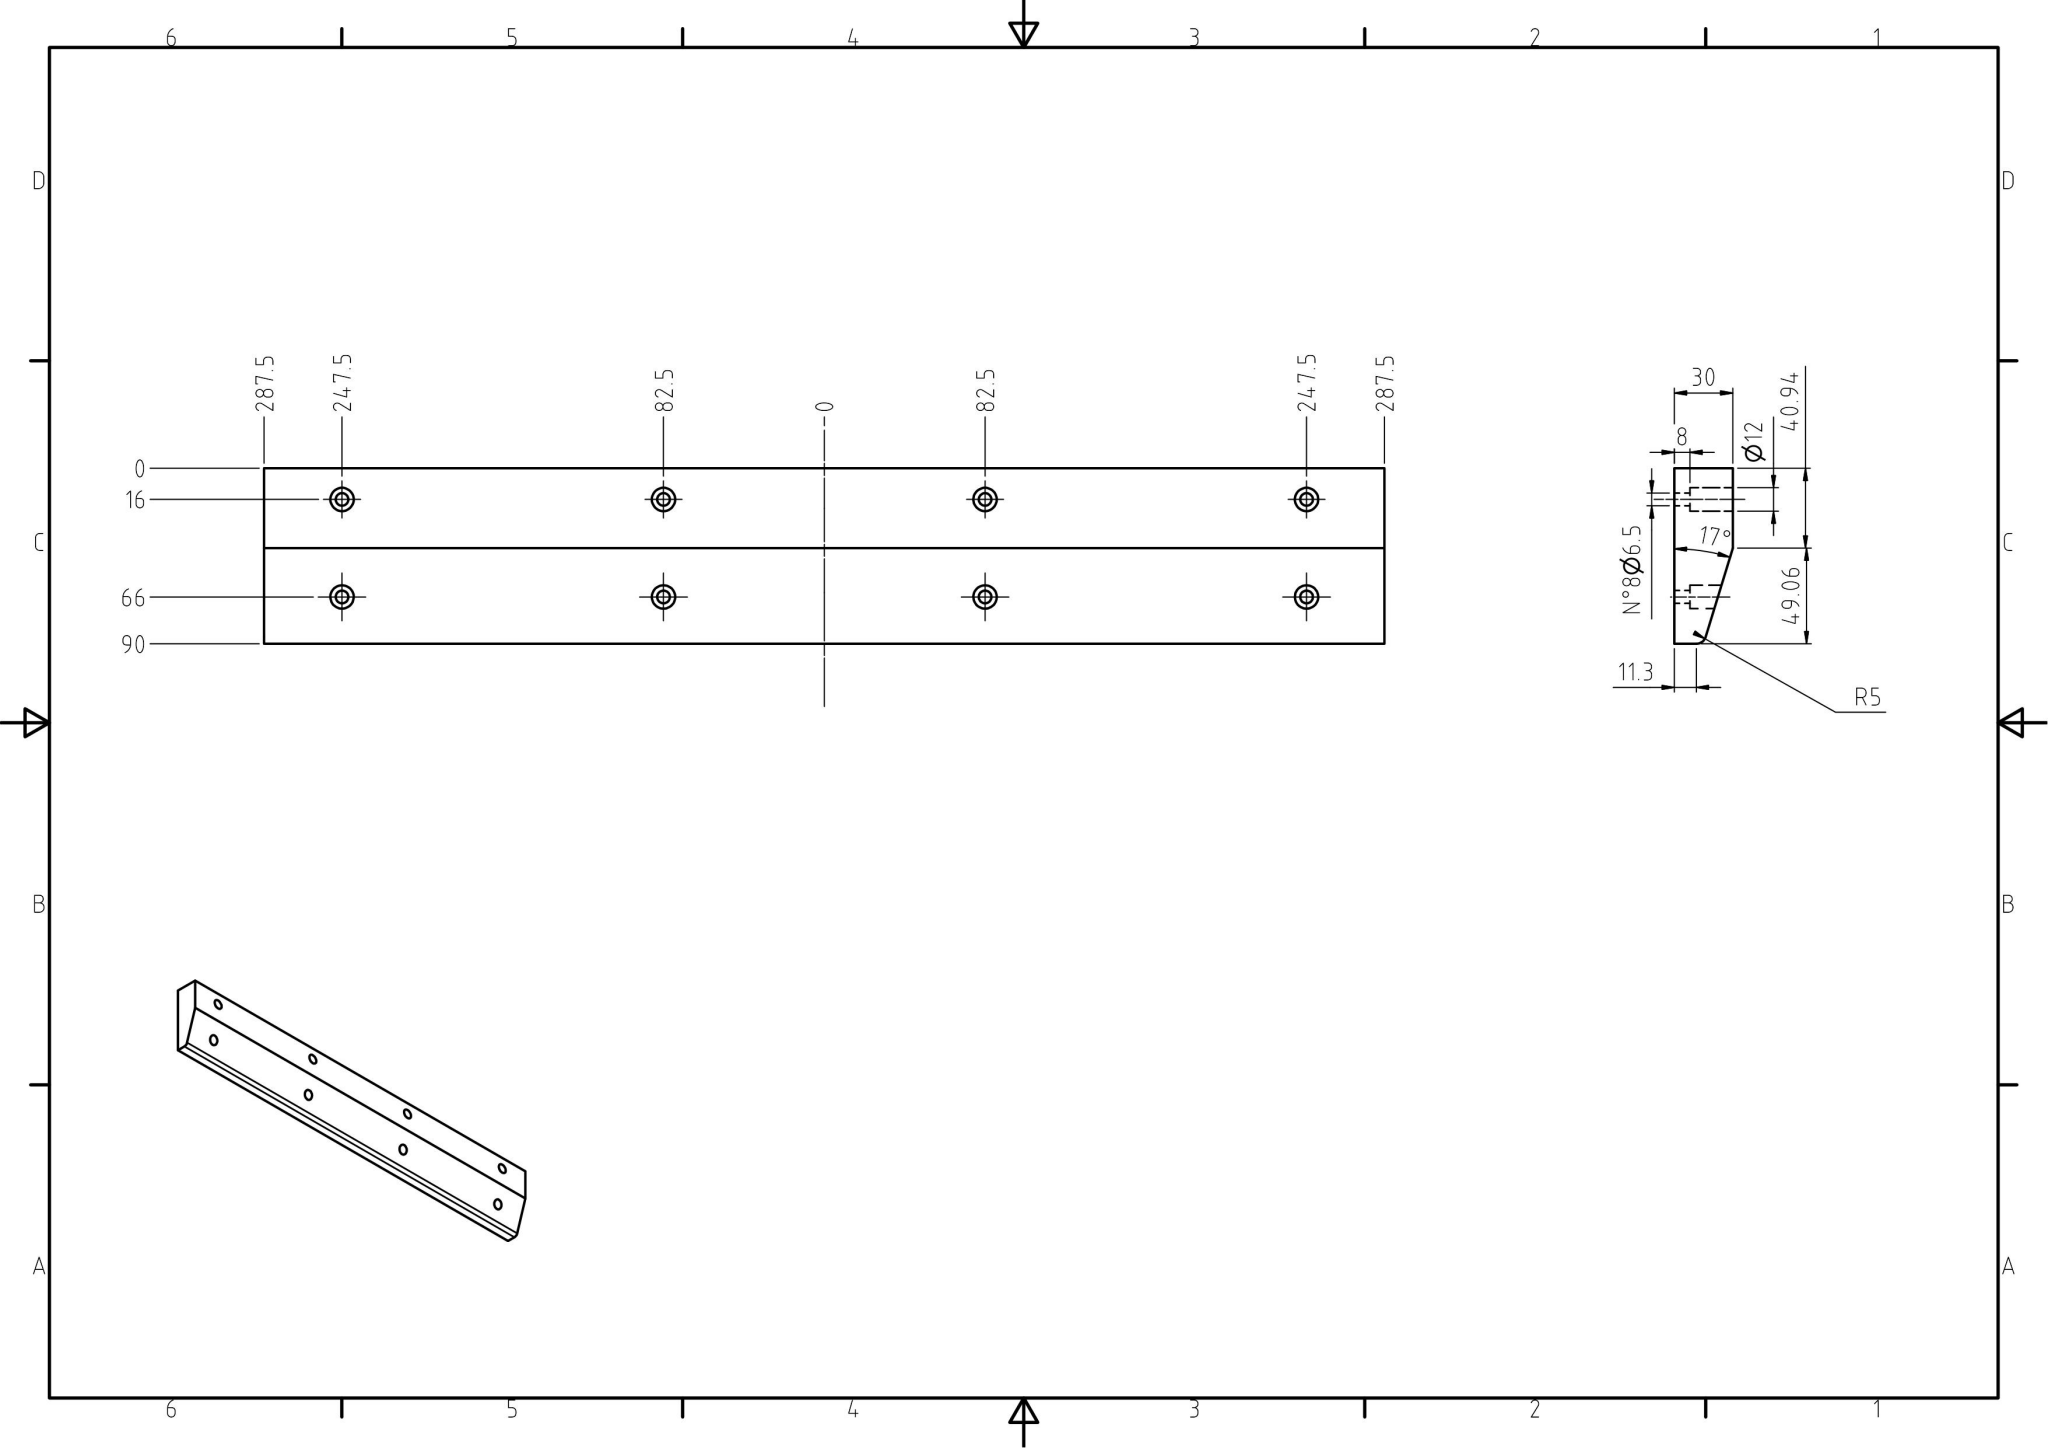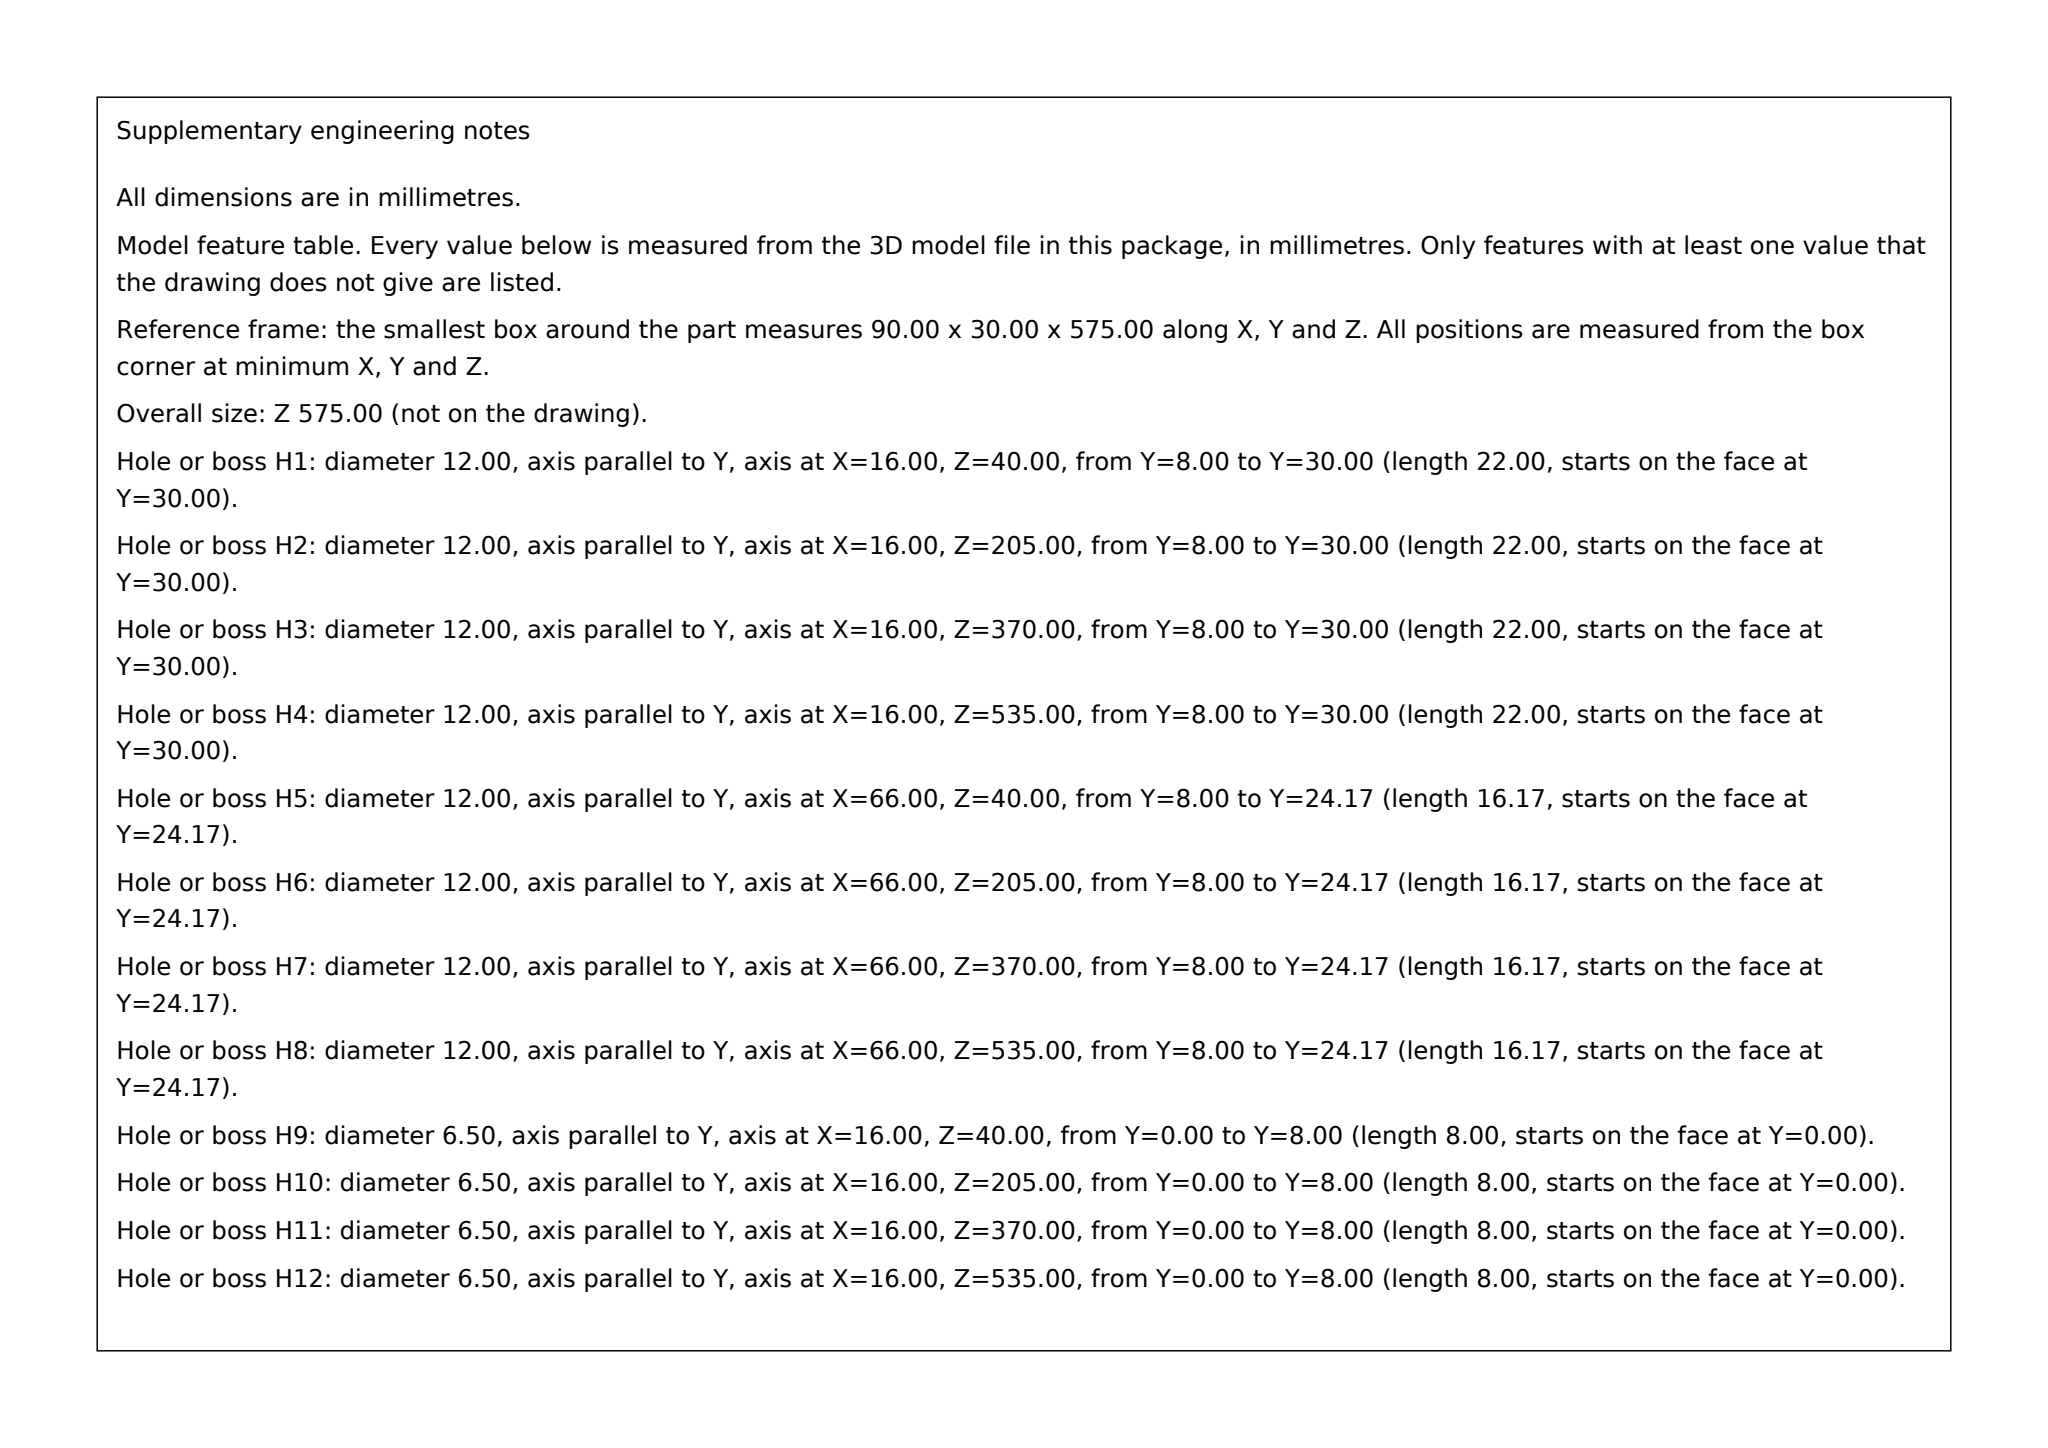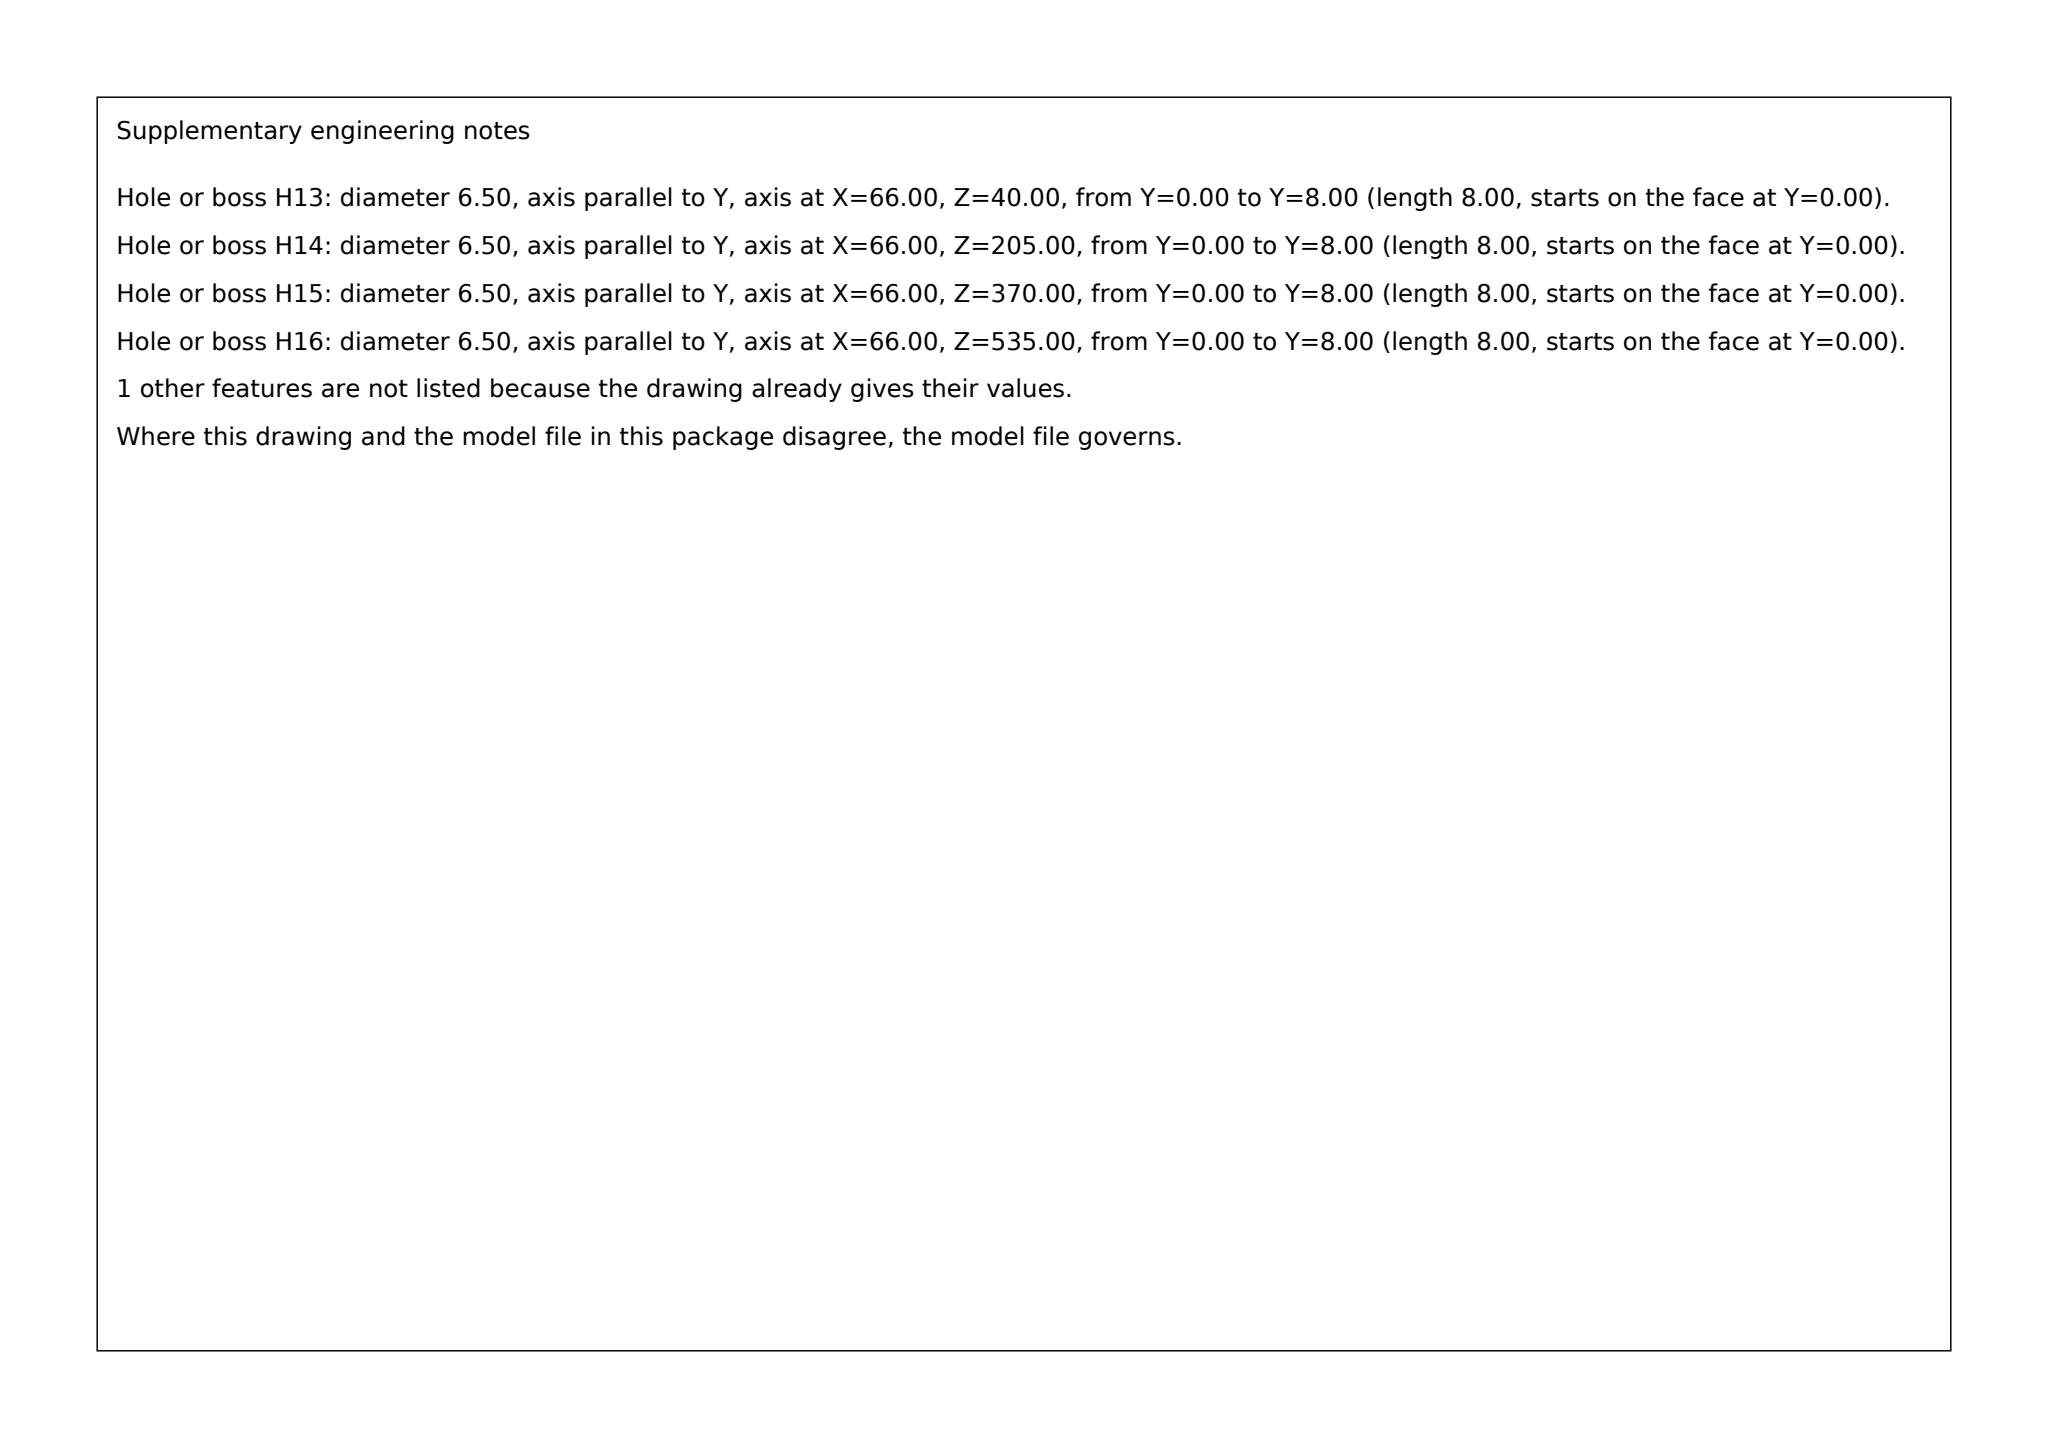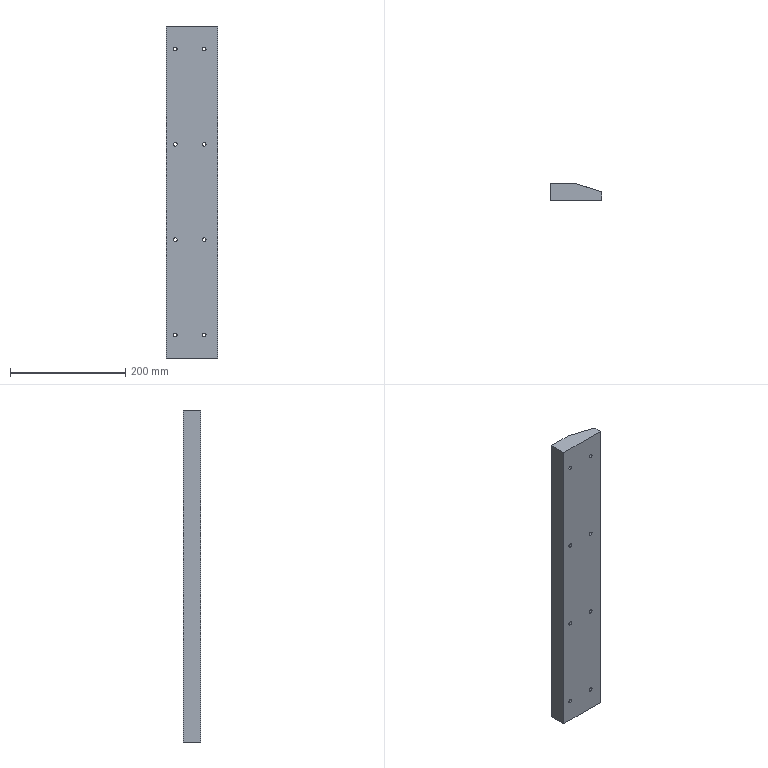Part | SolidWorks | mm | 1 solid | 49 faces | box 90 x 30 x 575 mm | volume 1320875 mm3 | cylinder 34 | plane 15 | commonest cylinder face diameters 6.5 x16 12 x16 10 x2